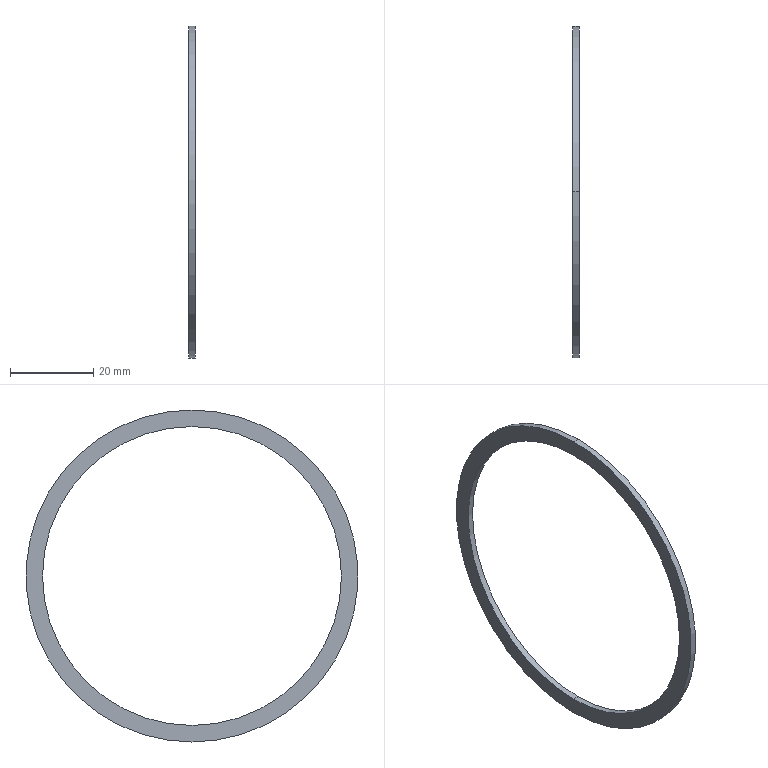Component | SolidWorks | 25SealRing-1 | 1 solid | 6 faces | box 1.5 x 80 x 80 mm | volume 1433 mm3 | cylinder 4 | plane 2 | commonest cylinder face diameters 72 x2 80 x2
build123d program:
from build123d import *

# Parameters (mm, degrees)
SKETCH1_R           = 40
SKETCH1_R_2         = 36
BOSS_EXTRUDE1_DEPTH = 1.5


with BuildPart() as part:
    # Sketch1 → Boss-Extrude1 (new body)
    with BuildSketch(Plane(origin=(0, 0, 0), x_dir=(0, 0, -1), z_dir=(1, 0, 0))):
        Circle(SKETCH1_R)
        Circle(SKETCH1_R_2, mode=Mode.SUBTRACT)
    extrude(amount=BOSS_EXTRUDE1_DEPTH)


solid = part.part

# Placed as in the assembly
solid = solid.moved(Location((-65.043, 1.776, 250), (0, 0, 0)))
STEP:
#1=CARTESIAN_POINT('',(-2.502,0.06992,11.26));
#2=VERTEX_POINT('',#1);
#3=CARTESIAN_POINT('',(-2.502,0.06992,8.425));
#4=VERTEX_POINT('',#3);
#5=CARTESIAN_POINT('',(-2.502,0.06992,9.843));
#6=DIRECTION('',(1.,0.,0.));
#7=DIRECTION('',(0.,0.,-1.));
#8=AXIS2_PLACEMENT_3D('',#5,#6,#7);
#9=CIRCLE('',#8,1.417);
#10=EDGE_CURVE('',#2,#4,#9,.T.);
#11=ORIENTED_EDGE('',*,*,#10,.T.);
#12=CARTESIAN_POINT('',(-2.561,0.06992,8.425));
#13=VERTEX_POINT('',#12);
#14=CARTESIAN_POINT('',(-2.502,0.06992,8.425));
#15=DIRECTION('',(-1.,0.,0.));
#16=VECTOR('',#15,39.37);
#17=LINE('',#14,#16);
#18=EDGE_CURVE('',#4,#13,#17,.T.);
#19=ORIENTED_EDGE('',*,*,#18,.T.);
#20=CARTESIAN_POINT('',(-2.561,0.06992,11.26));
#21=VERTEX_POINT('',#20);
#22=CARTESIAN_POINT('',(-2.561,0.06992,9.843));
#23=DIRECTION('',(1.,0.,0.));
#24=DIRECTION('',(0.,0.,-1.));
#25=AXIS2_PLACEMENT_3D('',#22,#23,#24);
#26=CIRCLE('',#25,1.417);
#27=EDGE_CURVE('',#21,#13,#26,.T.);
#28=ORIENTED_EDGE('',*,*,#27,.F.);
#29=CARTESIAN_POINT('',(-2.502,0.06992,11.26));
#30=DIRECTION('',(-1.,0.,0.));
#31=VECTOR('',#30,39.37);
#32=LINE('',#29,#31);
#33=EDGE_CURVE('',#2,#21,#32,.T.);
#34=ORIENTED_EDGE('',*,*,#33,.F.);
#35=EDGE_LOOP('',(#11,#19,#28,#34));
#36=FACE_OUTER_BOUND('',#35,.T.);
#37=CARTESIAN_POINT('',(-2.502,0.06992,9.843));
#38=DIRECTION('',(-1.,0.,0.));
#39=DIRECTION('',(0.,0.,1.));
#40=AXIS2_PLACEMENT_3D('',#37,#38,#39);
#41=CYLINDRICAL_SURFACE('',#40,1.417);
#42=ADVANCED_FACE('',(#36),#41,.F.);
#43=CARTESIAN_POINT('',(-2.502,0.06992,8.268));
#44=VERTEX_POINT('',#43);
#45=CARTESIAN_POINT('',(-2.502,0.06992,11.417));
#46=VERTEX_POINT('',#45);
#47=CARTESIAN_POINT('',(-2.502,0.06992,9.843));
#48=DIRECTION('',(1.,0.,0.));
#49=DIRECTION('',(0.,0.,-1.));
#50=AXIS2_PLACEMENT_3D('',#47,#48,#49);
#51=CIRCLE('',#50,1.575);
#52=EDGE_CURVE('',#44,#46,#51,.T.);
#53=ORIENTED_EDGE('',*,*,#52,.F.);
#54=CARTESIAN_POINT('',(-2.561,0.06992,8.268));
#55=VERTEX_POINT('',#54);
#56=CARTESIAN_POINT('',(-2.502,0.06992,8.268));
#57=DIRECTION('',(-1.,0.,0.));
#58=VECTOR('',#57,39.37);
#59=LINE('',#56,#58);
#60=EDGE_CURVE('',#44,#55,#59,.T.);
#61=ORIENTED_EDGE('',*,*,#60,.T.);
#62=CARTESIAN_POINT('',(-2.561,0.06992,11.417));
#63=VERTEX_POINT('',#62);
#64=CARTESIAN_POINT('',(-2.561,0.06992,9.843));
#65=DIRECTION('',(1.,0.,0.));
#66=DIRECTION('',(0.,0.,-1.));
#67=AXIS2_PLACEMENT_3D('',#64,#65,#66);
#68=CIRCLE('',#67,1.575);
#69=EDGE_CURVE('',#55,#63,#68,.T.);
#70=ORIENTED_EDGE('',*,*,#69,.T.);
#71=CARTESIAN_POINT('',(-2.502,0.06992,11.417));
#72=DIRECTION('',(-1.,0.,0.));
#73=VECTOR('',#72,39.37);
#74=LINE('',#71,#73);
#75=EDGE_CURVE('',#46,#63,#74,.T.);
#76=ORIENTED_EDGE('',*,*,#75,.F.);
#77=EDGE_LOOP('',(#53,#61,#70,#76));
#78=FACE_OUTER_BOUND('',#77,.T.);
#79=CARTESIAN_POINT('',(-2.502,0.06992,9.843));
#80=DIRECTION('',(-1.,0.,0.));
#81=DIRECTION('',(0.,0.,1.));
#82=AXIS2_PLACEMENT_3D('',#79,#80,#81);
#83=CYLINDRICAL_SURFACE('',#82,1.575);
#84=ADVANCED_FACE('',(#78),#83,.T.);
#85=CARTESIAN_POINT('',(-2.502,0.06992,9.843));
#86=DIRECTION('',(1.,0.,0.));
#87=DIRECTION('',(0.,0.,-1.));
#88=AXIS2_PLACEMENT_3D('',#85,#86,#87);
#89=CIRCLE('',#88,1.575);
#90=EDGE_CURVE('',#46,#44,#89,.T.);
#91=ORIENTED_EDGE('',*,*,#90,.T.);
#92=ORIENTED_EDGE('',*,*,#52,.T.);
#93=EDGE_LOOP('',(#91,#92));
#94=FACE_OUTER_BOUND('',#93,.T.);
#95=ORIENTED_EDGE('',*,*,#10,.F.);
#96=CARTESIAN_POINT('',(-2.502,0.06992,9.843));
#97=DIRECTION('',(1.,0.,0.));
#98=DIRECTION('',(0.,0.,-1.));
#99=AXIS2_PLACEMENT_3D('',#96,#97,#98);
#100=CIRCLE('',#99,1.417);
#101=EDGE_CURVE('',#4,#2,#100,.T.);
#102=ORIENTED_EDGE('',*,*,#101,.F.);
#103=EDGE_LOOP('',(#95,#102));
#104=FACE_BOUND('',#103,.T.);
#105=CARTESIAN_POINT('',(-2.502,0.06992,9.843));
#106=DIRECTION('',(1.,0.,0.));
#107=DIRECTION('',(0.,0.,-1.));
#108=AXIS2_PLACEMENT_3D('',#105,#106,#107);
#109=PLANE('',#108);
#110=ADVANCED_FACE('',(#94,#104),#109,.T.);
#111=CARTESIAN_POINT('',(-2.561,0.06992,9.843));
#112=DIRECTION('',(1.,0.,0.));
#113=DIRECTION('',(0.,0.,-1.));
#114=AXIS2_PLACEMENT_3D('',#111,#112,#113);
#115=CIRCLE('',#114,1.575);
#116=EDGE_CURVE('',#63,#55,#115,.T.);
#117=ORIENTED_EDGE('',*,*,#116,.F.);
#118=ORIENTED_EDGE('',*,*,#69,.F.);
#119=EDGE_LOOP('',(#117,#118));
#120=FACE_OUTER_BOUND('',#119,.T.);
#121=ORIENTED_EDGE('',*,*,#27,.T.);
#122=CARTESIAN_POINT('',(-2.561,0.06992,9.843));
#123=DIRECTION('',(1.,0.,0.));
#124=DIRECTION('',(0.,0.,-1.));
#125=AXIS2_PLACEMENT_3D('',#122,#123,#124);
#126=CIRCLE('',#125,1.417);
#127=EDGE_CURVE('',#13,#21,#126,.T.);
#128=ORIENTED_EDGE('',*,*,#127,.T.);
#129=EDGE_LOOP('',(#121,#128));
#130=FACE_BOUND('',#129,.T.);
#131=CARTESIAN_POINT('',(-2.561,0.06992,9.843));
#132=DIRECTION('',(1.,0.,0.));
#133=DIRECTION('',(0.,0.,-1.));
#134=AXIS2_PLACEMENT_3D('',#131,#132,#133);
#135=PLANE('',#134);
#136=ADVANCED_FACE('',(#120,#130),#135,.F.);
#137=ORIENTED_EDGE('',*,*,#60,.F.);
#138=ORIENTED_EDGE('',*,*,#90,.F.);
#139=ORIENTED_EDGE('',*,*,#75,.T.);
#140=ORIENTED_EDGE('',*,*,#116,.T.);
#141=EDGE_LOOP('',(#137,#138,#139,#140));
#142=FACE_OUTER_BOUND('',#141,.T.);
#143=CARTESIAN_POINT('',(-2.502,0.06992,9.843));
#144=DIRECTION('',(-1.,0.,0.));
#145=DIRECTION('',(0.,0.,1.));
#146=AXIS2_PLACEMENT_3D('',#143,#144,#145);
#147=CYLINDRICAL_SURFACE('',#146,1.575);
#148=ADVANCED_FACE('',(#142),#147,.T.);
#149=ORIENTED_EDGE('',*,*,#18,.F.);
#150=ORIENTED_EDGE('',*,*,#101,.T.);
#151=ORIENTED_EDGE('',*,*,#33,.T.);
#152=ORIENTED_EDGE('',*,*,#127,.F.);
#153=EDGE_LOOP('',(#149,#150,#151,#152));
#154=FACE_OUTER_BOUND('',#153,.T.);
#155=CARTESIAN_POINT('',(-2.502,0.06992,9.843));
#156=DIRECTION('',(-1.,0.,0.));
#157=DIRECTION('',(0.,0.,1.));
#158=AXIS2_PLACEMENT_3D('',#155,#156,#157);
#159=CYLINDRICAL_SURFACE('',#158,1.417);
#160=ADVANCED_FACE('',(#154),#159,.F.);
#161=CLOSED_SHELL('',(#42,#84,#110,#136,#148,#160));
#162=MANIFOLD_SOLID_BREP('',#161);
#163=CARTESIAN_POINT('',(0.,0.,0.));
#164=DIRECTION('',(0.,0.,1.));
#165=DIRECTION('',(1.,0.,0.));
#166=AXIS2_PLACEMENT_3D('',#163,#164,#165);
#167=(LENGTH_UNIT()NAMED_UNIT(*)SI_UNIT($,.METRE.));
#168=LENGTH_MEASURE_WITH_UNIT(LENGTH_MEASURE(0.0254),#167);
#169=DIMENSIONAL_EXPONENTS(1.,0.,0.,0.,0.,0.,0.);
#170=(CONVERSION_BASED_UNIT('',#168)LENGTH_UNIT()NAMED_UNIT(#169));
#171=UNCERTAINTY_MEASURE_WITH_UNIT(LENGTH_MEASURE(0.00001),#170,'','');
#172=(NAMED_UNIT(*)PLANE_ANGLE_UNIT()SI_UNIT($,.RADIAN.));
#173=(NAMED_UNIT(*)SI_UNIT($,.STERADIAN.)SOLID_ANGLE_UNIT());
#174=(GEOMETRIC_REPRESENTATION_CONTEXT(3)GLOBAL_UNCERTAINTY_ASSIGNED_CONTEXT((#171))GLOBAL_UNIT_ASSIGNED_CONTEXT((#170,#172,#173))REPRESENTATION_CONTEXT('',''));
#175=ADVANCED_BREP_SHAPE_REPRESENTATION('',(#162,#166),#174);
#176=COLOUR_RGB('',0.7922,0.8196,0.9333);
#177=FILL_AREA_STYLE_COLOUR('',#176);
#178=FILL_AREA_STYLE('',(#177));
#179=SURFACE_STYLE_FILL_AREA(#178);
#180=SURFACE_SIDE_STYLE('',(#179));
#181=SURFACE_STYLE_USAGE(.BOTH.,#180);
#182=PRESENTATION_STYLE_ASSIGNMENT((#181));
#183=STYLED_ITEM('',(#182),#162);
#184=(LENGTH_UNIT()NAMED_UNIT(*)SI_UNIT($,.METRE.));
#185=LENGTH_MEASURE_WITH_UNIT(LENGTH_MEASURE(0.0254),#184);
#186=DIMENSIONAL_EXPONENTS(1.,0.,0.,0.,0.,0.,0.);
#187=(CONVERSION_BASED_UNIT('',#185)LENGTH_UNIT()NAMED_UNIT(#186));
#188=UNCERTAINTY_MEASURE_WITH_UNIT(LENGTH_MEASURE(0.00001),#187,'','');
#189=(NAMED_UNIT(*)PLANE_ANGLE_UNIT()SI_UNIT($,.RADIAN.));
#190=(NAMED_UNIT(*)SI_UNIT($,.STERADIAN.)SOLID_ANGLE_UNIT());
#191=(GEOMETRIC_REPRESENTATION_CONTEXT(3)GLOBAL_UNCERTAINTY_ASSIGNED_CONTEXT((#188))GLOBAL_UNIT_ASSIGNED_CONTEXT((#187,#189,#190))REPRESENTATION_CONTEXT('',''));
#192=MECHANICAL_DESIGN_GEOMETRIC_PRESENTATION_REPRESENTATION('',(#183),#191);
#193=PRESENTATION_LAYER_ASSIGNMENT('','',(#183));